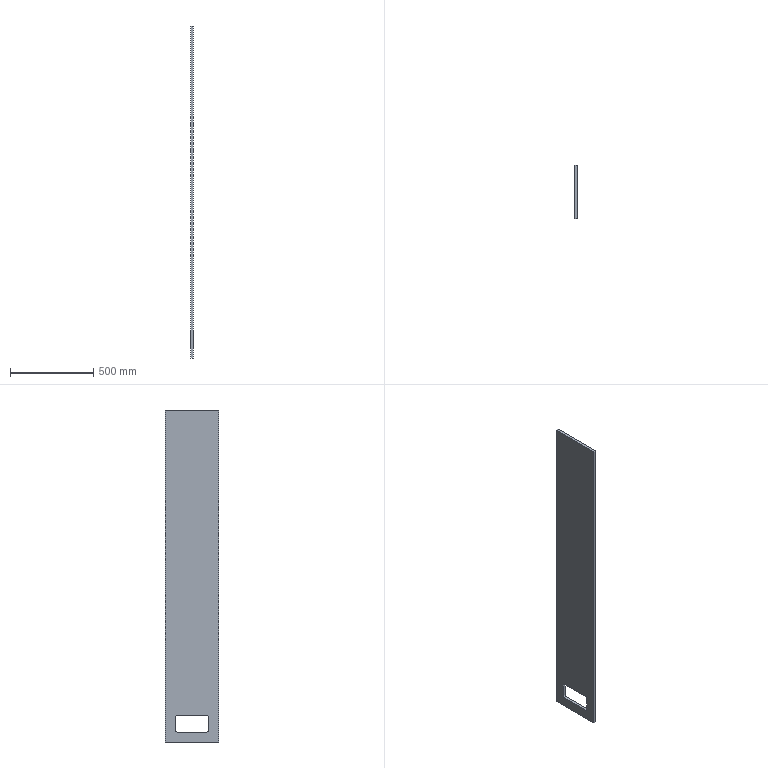Component | NX | CH3404_5-1 | 1 solid | 14 faces | box 16 x 321 x 2000 mm | volume 9953373 mm3 | plane 10 | cylinder 4 | commonest cylinder face diameters 20 x4
STEP:
#1=CARTESIAN_POINT('',(0.,0.,0.));
#2=DIRECTION('',(0.,0.,1.));
#3=DIRECTION('',(1.,0.,0.));
#4=AXIS2_PLACEMENT_3D('',#1,#2,#3);
#5=CARTESIAN_POINT('',(295.,-100.,-155.));
#6=VERTEX_POINT('',#5);
#7=CARTESIAN_POINT('',(295.,-100.,-75.));
#8=VERTEX_POINT('',#7);
#9=CARTESIAN_POINT('',(295.,-100.,-165.));
#10=DIRECTION('',(0.,0.,1.));
#11=VECTOR('',#10,1.);
#12=LINE('',#9,#11);
#13=CARTESIAN_POINT('',(295.,-100.,-165.));
#14=DIRECTION('',(0.,-1.,0.));
#15=DIRECTION('',(0.,0.,-1.));
#16=AXIS2_PLACEMENT_3D('',#13,#14,#15);
#17=PLANE('',#16);
#18=CARTESIAN_POINT('',(0.,0.));
#19=DIRECTION('',(-1.,0.));
#20=VECTOR('',#19,1.);
#21=LINE('',#18,#20);
#22=(GEOMETRIC_REPRESENTATION_CONTEXT(2)PARAMETRIC_REPRESENTATION_CONTEXT()REPRESENTATION_CONTEXT('',''));
#23=DEFINITIONAL_REPRESENTATION('',(#21),#22);
#24=PCURVE('',#17,#23);
#25=CARTESIAN_POINT('',(295.,0.,-225.));
#26=DIRECTION('',(1.,0.,0.));
#27=DIRECTION('',(0.,0.,-1.));
#28=AXIS2_PLACEMENT_3D('',#25,#26,#27);
#29=PLANE('',#28);
#30=CARTESIAN_POINT('',(-60.,-100.));
#31=DIRECTION('',(-1.,0.));
#32=VECTOR('',#31,1.);
#33=LINE('',#30,#32);
#34=(GEOMETRIC_REPRESENTATION_CONTEXT(2)PARAMETRIC_REPRESENTATION_CONTEXT()REPRESENTATION_CONTEXT('',''));
#35=DEFINITIONAL_REPRESENTATION('',(#33),#34);
#36=PCURVE('',#29,#35);
#37=SURFACE_CURVE('',#12,(#24,#36),.PCURVE_S1.);
#38=EDGE_CURVE('',#6,#8,#37,.T.);
#39=ORIENTED_EDGE('',*,*,#38,.F.);
#40=CARTESIAN_POINT('',(279.,-100.,-155.));
#41=VERTEX_POINT('',#40);
#42=CARTESIAN_POINT('',(279.,-100.,-155.));
#43=DIRECTION('',(-1.,0.,0.));
#44=VECTOR('',#43,1.);
#45=LINE('',#42,#44);
#46=CARTESIAN_POINT('',(-10.,-16.));
#47=DIRECTION('',(0.,-1.));
#48=VECTOR('',#47,1.);
#49=LINE('',#46,#48);
#50=(GEOMETRIC_REPRESENTATION_CONTEXT(2)PARAMETRIC_REPRESENTATION_CONTEXT()REPRESENTATION_CONTEXT('',''));
#51=DEFINITIONAL_REPRESENTATION('',(#49),#50);
#52=PCURVE('',#17,#51);
#53=CARTESIAN_POINT('',(295.,-90.,-155.));
#54=DIRECTION('',(1.,0.,0.));
#55=DIRECTION('',(0.,0.,-1.));
#56=AXIS2_PLACEMENT_3D('',#53,#54,#55);
#57=CYLINDRICAL_SURFACE('',#56,10.);
#58=CARTESIAN_POINT('',(4.712,-16.));
#59=DIRECTION('',(0.,-1.));
#60=VECTOR('',#59,1.);
#61=LINE('',#58,#60);
#62=(GEOMETRIC_REPRESENTATION_CONTEXT(2)PARAMETRIC_REPRESENTATION_CONTEXT()REPRESENTATION_CONTEXT('',''));
#63=DEFINITIONAL_REPRESENTATION('',(#61),#62);
#64=PCURVE('',#57,#63);
#65=SURFACE_CURVE('',#45,(#52,#64),.PCURVE_S1.);
#66=EDGE_CURVE('',#6,#41,#65,.T.);
#67=ORIENTED_EDGE('',*,*,#66,.T.);
#68=CARTESIAN_POINT('',(279.,-100.,-75.));
#69=VERTEX_POINT('',#68);
#70=CARTESIAN_POINT('',(279.,-100.,-165.));
#71=DIRECTION('',(0.,0.,1.));
#72=VECTOR('',#71,1.);
#73=LINE('',#70,#72);
#74=CARTESIAN_POINT('',(0.,-16.));
#75=DIRECTION('',(-1.,0.));
#76=VECTOR('',#75,1.);
#77=LINE('',#74,#76);
#78=(GEOMETRIC_REPRESENTATION_CONTEXT(2)PARAMETRIC_REPRESENTATION_CONTEXT()REPRESENTATION_CONTEXT('',''));
#79=DEFINITIONAL_REPRESENTATION('',(#77),#78);
#80=PCURVE('',#17,#79);
#81=CARTESIAN_POINT('',(279.,0.,-225.));
#82=DIRECTION('',(1.,0.,0.));
#83=DIRECTION('',(0.,0.,-1.));
#84=AXIS2_PLACEMENT_3D('',#81,#82,#83);
#85=PLANE('',#84);
#86=CARTESIAN_POINT('',(-60.,-100.));
#87=DIRECTION('',(-1.,0.));
#88=VECTOR('',#87,1.);
#89=LINE('',#86,#88);
#90=(GEOMETRIC_REPRESENTATION_CONTEXT(2)PARAMETRIC_REPRESENTATION_CONTEXT()REPRESENTATION_CONTEXT('',''));
#91=DEFINITIONAL_REPRESENTATION('',(#89),#90);
#92=PCURVE('',#85,#91);
#93=SURFACE_CURVE('',#73,(#80,#92),.PCURVE_S1.);
#94=EDGE_CURVE('',#41,#69,#93,.T.);
#95=ORIENTED_EDGE('',*,*,#94,.T.);
#96=CARTESIAN_POINT('',(295.,-100.,-75.));
#97=DIRECTION('',(1.,0.,0.));
#98=VECTOR('',#97,1.);
#99=LINE('',#96,#98);
#100=CARTESIAN_POINT('',(-90.,0.));
#101=DIRECTION('',(0.,1.));
#102=VECTOR('',#101,1.);
#103=LINE('',#100,#102);
#104=(GEOMETRIC_REPRESENTATION_CONTEXT(2)PARAMETRIC_REPRESENTATION_CONTEXT()REPRESENTATION_CONTEXT('',''));
#105=DEFINITIONAL_REPRESENTATION('',(#103),#104);
#106=PCURVE('',#17,#105);
#107=CARTESIAN_POINT('',(295.,-90.,-75.));
#108=DIRECTION('',(1.,0.,0.));
#109=DIRECTION('',(0.,0.,-1.));
#110=AXIS2_PLACEMENT_3D('',#107,#108,#109);
#111=CYLINDRICAL_SURFACE('',#110,10.);
#112=CARTESIAN_POINT('',(4.712,0.));
#113=DIRECTION('',(0.,1.));
#114=VECTOR('',#113,1.);
#115=LINE('',#112,#114);
#116=(GEOMETRIC_REPRESENTATION_CONTEXT(2)PARAMETRIC_REPRESENTATION_CONTEXT()REPRESENTATION_CONTEXT('',''));
#117=DEFINITIONAL_REPRESENTATION('',(#115),#116);
#118=PCURVE('',#111,#117);
#119=SURFACE_CURVE('',#99,(#106,#118),.PCURVE_S1.);
#120=EDGE_CURVE('',#69,#8,#119,.T.);
#121=ORIENTED_EDGE('',*,*,#120,.T.);
#122=EDGE_LOOP('',(#39,#67,#95,#121));
#123=FACE_BOUND('',#122,.T.);
#124=ADVANCED_FACE('',(#123),#17,.F.);
#125=CARTESIAN_POINT('',(295.,-90.,-65.));
#126=VERTEX_POINT('',#125);
#127=CARTESIAN_POINT('',(295.,90.,-65.));
#128=VERTEX_POINT('',#127);
#129=CARTESIAN_POINT('',(295.,-100.,-65.));
#130=DIRECTION('',(0.,1.,0.));
#131=VECTOR('',#130,1.);
#132=LINE('',#129,#131);
#133=CARTESIAN_POINT('',(295.,-100.,-65.));
#134=DIRECTION('',(0.,0.,1.));
#135=DIRECTION('',(1.,0.,0.));
#136=AXIS2_PLACEMENT_3D('',#133,#134,#135);
#137=PLANE('',#136);
#138=CARTESIAN_POINT('',(0.,0.));
#139=DIRECTION('',(0.,1.));
#140=VECTOR('',#139,1.);
#141=LINE('',#138,#140);
#142=(GEOMETRIC_REPRESENTATION_CONTEXT(2)PARAMETRIC_REPRESENTATION_CONTEXT()REPRESENTATION_CONTEXT('',''));
#143=DEFINITIONAL_REPRESENTATION('',(#141),#142);
#144=PCURVE('',#137,#143);
#145=CARTESIAN_POINT('',(-160.,-100.));
#146=DIRECTION('',(0.,1.));
#147=VECTOR('',#146,1.);
#148=LINE('',#145,#147);
#149=(GEOMETRIC_REPRESENTATION_CONTEXT(2)PARAMETRIC_REPRESENTATION_CONTEXT()REPRESENTATION_CONTEXT('',''));
#150=DEFINITIONAL_REPRESENTATION('',(#148),#149);
#151=PCURVE('',#29,#150);
#152=SURFACE_CURVE('',#132,(#144,#151),.PCURVE_S1.);
#153=EDGE_CURVE('',#126,#128,#152,.T.);
#154=ORIENTED_EDGE('',*,*,#153,.F.);
#155=CARTESIAN_POINT('',(279.,-90.,-65.));
#156=VERTEX_POINT('',#155);
#157=CARTESIAN_POINT('',(279.,-90.,-65.));
#158=DIRECTION('',(-1.,0.,0.));
#159=VECTOR('',#158,1.);
#160=LINE('',#157,#159);
#161=CARTESIAN_POINT('',(-16.,10.));
#162=DIRECTION('',(-1.,0.));
#163=VECTOR('',#162,1.);
#164=LINE('',#161,#163);
#165=(GEOMETRIC_REPRESENTATION_CONTEXT(2)PARAMETRIC_REPRESENTATION_CONTEXT()REPRESENTATION_CONTEXT('',''));
#166=DEFINITIONAL_REPRESENTATION('',(#164),#165);
#167=PCURVE('',#137,#166);
#168=CARTESIAN_POINT('',(3.142,-16.));
#169=DIRECTION('',(0.,-1.));
#170=VECTOR('',#169,1.);
#171=LINE('',#168,#170);
#172=(GEOMETRIC_REPRESENTATION_CONTEXT(2)PARAMETRIC_REPRESENTATION_CONTEXT()REPRESENTATION_CONTEXT('',''));
#173=DEFINITIONAL_REPRESENTATION('',(#171),#172);
#174=PCURVE('',#111,#173);
#175=SURFACE_CURVE('',#160,(#167,#174),.PCURVE_S1.);
#176=EDGE_CURVE('',#126,#156,#175,.T.);
#177=ORIENTED_EDGE('',*,*,#176,.T.);
#178=CARTESIAN_POINT('',(279.,90.,-65.));
#179=VERTEX_POINT('',#178);
#180=CARTESIAN_POINT('',(279.,-100.,-65.));
#181=DIRECTION('',(0.,1.,0.));
#182=VECTOR('',#181,1.);
#183=LINE('',#180,#182);
#184=CARTESIAN_POINT('',(-16.,0.));
#185=DIRECTION('',(0.,1.));
#186=VECTOR('',#185,1.);
#187=LINE('',#184,#186);
#188=(GEOMETRIC_REPRESENTATION_CONTEXT(2)PARAMETRIC_REPRESENTATION_CONTEXT()REPRESENTATION_CONTEXT('',''));
#189=DEFINITIONAL_REPRESENTATION('',(#187),#188);
#190=PCURVE('',#137,#189);
#191=CARTESIAN_POINT('',(-160.,-100.));
#192=DIRECTION('',(0.,1.));
#193=VECTOR('',#192,1.);
#194=LINE('',#191,#193);
#195=(GEOMETRIC_REPRESENTATION_CONTEXT(2)PARAMETRIC_REPRESENTATION_CONTEXT()REPRESENTATION_CONTEXT('',''));
#196=DEFINITIONAL_REPRESENTATION('',(#194),#195);
#197=PCURVE('',#85,#196);
#198=SURFACE_CURVE('',#183,(#190,#197),.PCURVE_S1.);
#199=EDGE_CURVE('',#156,#179,#198,.T.);
#200=ORIENTED_EDGE('',*,*,#199,.T.);
#201=CARTESIAN_POINT('',(295.,90.,-65.));
#202=DIRECTION('',(1.,0.,0.));
#203=VECTOR('',#202,1.);
#204=LINE('',#201,#203);
#205=CARTESIAN_POINT('',(0.,190.));
#206=DIRECTION('',(1.,0.));
#207=VECTOR('',#206,1.);
#208=LINE('',#205,#207);
#209=(GEOMETRIC_REPRESENTATION_CONTEXT(2)PARAMETRIC_REPRESENTATION_CONTEXT()REPRESENTATION_CONTEXT('',''));
#210=DEFINITIONAL_REPRESENTATION('',(#208),#209);
#211=PCURVE('',#137,#210);
#212=CARTESIAN_POINT('',(295.,90.,-75.));
#213=DIRECTION('',(1.,0.,0.));
#214=DIRECTION('',(0.,0.,-1.));
#215=AXIS2_PLACEMENT_3D('',#212,#213,#214);
#216=CYLINDRICAL_SURFACE('',#215,10.);
#217=CARTESIAN_POINT('',(3.142,0.));
#218=DIRECTION('',(0.,1.));
#219=VECTOR('',#218,1.);
#220=LINE('',#217,#219);
#221=(GEOMETRIC_REPRESENTATION_CONTEXT(2)PARAMETRIC_REPRESENTATION_CONTEXT()REPRESENTATION_CONTEXT('',''));
#222=DEFINITIONAL_REPRESENTATION('',(#220),#221);
#223=PCURVE('',#216,#222);
#224=SURFACE_CURVE('',#204,(#211,#223),.PCURVE_S1.);
#225=EDGE_CURVE('',#179,#128,#224,.T.);
#226=ORIENTED_EDGE('',*,*,#225,.T.);
#227=EDGE_LOOP('',(#154,#177,#200,#226));
#228=FACE_BOUND('',#227,.T.);
#229=ADVANCED_FACE('',(#228),#137,.F.);
#230=CARTESIAN_POINT('',(279.,100.,-75.));
#231=VERTEX_POINT('',#230);
#232=CARTESIAN_POINT('',(279.,100.,-155.));
#233=VERTEX_POINT('',#232);
#234=CARTESIAN_POINT('',(279.,100.,-65.));
#235=DIRECTION('',(0.,0.,-1.));
#236=VECTOR('',#235,1.);
#237=LINE('',#234,#236);
#238=CARTESIAN_POINT('',(295.,100.,-65.));
#239=DIRECTION('',(0.,1.,0.));
#240=DIRECTION('',(0.,0.,1.));
#241=AXIS2_PLACEMENT_3D('',#238,#239,#240);
#242=PLANE('',#241);
#243=CARTESIAN_POINT('',(0.,-16.));
#244=DIRECTION('',(-1.,0.));
#245=VECTOR('',#244,1.);
#246=LINE('',#243,#245);
#247=(GEOMETRIC_REPRESENTATION_CONTEXT(2)PARAMETRIC_REPRESENTATION_CONTEXT()REPRESENTATION_CONTEXT('',''));
#248=DEFINITIONAL_REPRESENTATION('',(#246),#247);
#249=PCURVE('',#242,#248);
#250=CARTESIAN_POINT('',(-160.,100.));
#251=DIRECTION('',(1.,0.));
#252=VECTOR('',#251,1.);
#253=LINE('',#250,#252);
#254=(GEOMETRIC_REPRESENTATION_CONTEXT(2)PARAMETRIC_REPRESENTATION_CONTEXT()REPRESENTATION_CONTEXT('',''));
#255=DEFINITIONAL_REPRESENTATION('',(#253),#254);
#256=PCURVE('',#85,#255);
#257=SURFACE_CURVE('',#237,(#249,#256),.PCURVE_S1.);
#258=EDGE_CURVE('',#231,#233,#257,.T.);
#259=ORIENTED_EDGE('',*,*,#258,.T.);
#260=CARTESIAN_POINT('',(295.,100.,-155.));
#261=VERTEX_POINT('',#260);
#262=CARTESIAN_POINT('',(295.,100.,-155.));
#263=DIRECTION('',(1.,0.,0.));
#264=VECTOR('',#263,1.);
#265=LINE('',#262,#264);
#266=CARTESIAN_POINT('',(-90.,0.));
#267=DIRECTION('',(0.,1.));
#268=VECTOR('',#267,1.);
#269=LINE('',#266,#268);
#270=(GEOMETRIC_REPRESENTATION_CONTEXT(2)PARAMETRIC_REPRESENTATION_CONTEXT()REPRESENTATION_CONTEXT('',''));
#271=DEFINITIONAL_REPRESENTATION('',(#269),#270);
#272=PCURVE('',#242,#271);
#273=CARTESIAN_POINT('',(295.,90.,-155.));
#274=DIRECTION('',(1.,0.,0.));
#275=DIRECTION('',(0.,0.,-1.));
#276=AXIS2_PLACEMENT_3D('',#273,#274,#275);
#277=CYLINDRICAL_SURFACE('',#276,10.);
#278=CARTESIAN_POINT('',(1.571,0.));
#279=DIRECTION('',(0.,1.));
#280=VECTOR('',#279,1.);
#281=LINE('',#278,#280);
#282=(GEOMETRIC_REPRESENTATION_CONTEXT(2)PARAMETRIC_REPRESENTATION_CONTEXT()REPRESENTATION_CONTEXT('',''));
#283=DEFINITIONAL_REPRESENTATION('',(#281),#282);
#284=PCURVE('',#277,#283);
#285=SURFACE_CURVE('',#265,(#272,#284),.PCURVE_S1.);
#286=EDGE_CURVE('',#233,#261,#285,.T.);
#287=ORIENTED_EDGE('',*,*,#286,.T.);
#288=CARTESIAN_POINT('',(295.,100.,-75.));
#289=VERTEX_POINT('',#288);
#290=CARTESIAN_POINT('',(295.,100.,-65.));
#291=DIRECTION('',(0.,0.,-1.));
#292=VECTOR('',#291,1.);
#293=LINE('',#290,#292);
#294=CARTESIAN_POINT('',(0.,0.));
#295=DIRECTION('',(-1.,0.));
#296=VECTOR('',#295,1.);
#297=LINE('',#294,#296);
#298=(GEOMETRIC_REPRESENTATION_CONTEXT(2)PARAMETRIC_REPRESENTATION_CONTEXT()REPRESENTATION_CONTEXT('',''));
#299=DEFINITIONAL_REPRESENTATION('',(#297),#298);
#300=PCURVE('',#242,#299);
#301=CARTESIAN_POINT('',(-160.,100.));
#302=DIRECTION('',(1.,0.));
#303=VECTOR('',#302,1.);
#304=LINE('',#301,#303);
#305=(GEOMETRIC_REPRESENTATION_CONTEXT(2)PARAMETRIC_REPRESENTATION_CONTEXT()REPRESENTATION_CONTEXT('',''));
#306=DEFINITIONAL_REPRESENTATION('',(#304),#305);
#307=PCURVE('',#29,#306);
#308=SURFACE_CURVE('',#293,(#300,#307),.PCURVE_S1.);
#309=EDGE_CURVE('',#289,#261,#308,.T.);
#310=ORIENTED_EDGE('',*,*,#309,.F.);
#311=CARTESIAN_POINT('',(279.,100.,-75.));
#312=DIRECTION('',(-1.,0.,0.));
#313=VECTOR('',#312,1.);
#314=LINE('',#311,#313);
#315=CARTESIAN_POINT('',(-10.,-16.));
#316=DIRECTION('',(0.,-1.));
#317=VECTOR('',#316,1.);
#318=LINE('',#315,#317);
#319=(GEOMETRIC_REPRESENTATION_CONTEXT(2)PARAMETRIC_REPRESENTATION_CONTEXT()REPRESENTATION_CONTEXT('',''));
#320=DEFINITIONAL_REPRESENTATION('',(#318),#319);
#321=PCURVE('',#242,#320);
#322=CARTESIAN_POINT('',(1.571,-16.));
#323=DIRECTION('',(0.,-1.));
#324=VECTOR('',#323,1.);
#325=LINE('',#322,#324);
#326=(GEOMETRIC_REPRESENTATION_CONTEXT(2)PARAMETRIC_REPRESENTATION_CONTEXT()REPRESENTATION_CONTEXT('',''));
#327=DEFINITIONAL_REPRESENTATION('',(#325),#326);
#328=PCURVE('',#216,#327);
#329=SURFACE_CURVE('',#314,(#321,#328),.PCURVE_S1.);
#330=EDGE_CURVE('',#289,#231,#329,.T.);
#331=ORIENTED_EDGE('',*,*,#330,.T.);
#332=EDGE_LOOP('',(#259,#287,#310,#331));
#333=FACE_BOUND('',#332,.T.);
#334=ADVANCED_FACE('',(#333),#242,.F.);
#335=CARTESIAN_POINT('',(279.,-160.5,1775.));
#336=VERTEX_POINT('',#335);
#337=CARTESIAN_POINT('',(279.,-160.5,-225.));
#338=VERTEX_POINT('',#337);
#339=CARTESIAN_POINT('',(279.,-160.5,1775.));
#340=DIRECTION('',(0.,-0.,-1.));
#341=VECTOR('',#340,1.);
#342=LINE('',#339,#341);
#343=CARTESIAN_POINT('',(295.,-160.5,1775.));
#344=DIRECTION('',(0.,1.,-0.));
#345=DIRECTION('',(0.,0.,1.));
#346=AXIS2_PLACEMENT_3D('',#343,#344,#345);
#347=PLANE('',#346);
#348=CARTESIAN_POINT('',(0.,-16.));
#349=DIRECTION('',(-1.,0.));
#350=VECTOR('',#349,1.);
#351=LINE('',#348,#350);
#352=(GEOMETRIC_REPRESENTATION_CONTEXT(2)PARAMETRIC_REPRESENTATION_CONTEXT()REPRESENTATION_CONTEXT('',''));
#353=DEFINITIONAL_REPRESENTATION('',(#351),#352);
#354=PCURVE('',#347,#353);
#355=CARTESIAN_POINT('',(-2000.,-160.5));
#356=DIRECTION('',(1.,-0.));
#357=VECTOR('',#356,1.);
#358=LINE('',#355,#357);
#359=(GEOMETRIC_REPRESENTATION_CONTEXT(2)PARAMETRIC_REPRESENTATION_CONTEXT()REPRESENTATION_CONTEXT('',''));
#360=DEFINITIONAL_REPRESENTATION('',(#358),#359);
#361=PCURVE('',#85,#360);
#362=SURFACE_CURVE('',#342,(#354,#361),.PCURVE_S1.);
#363=EDGE_CURVE('',#336,#338,#362,.T.);
#364=ORIENTED_EDGE('',*,*,#363,.T.);
#365=CARTESIAN_POINT('',(295.,-160.5,-225.));
#366=VERTEX_POINT('',#365);
#367=CARTESIAN_POINT('',(295.,-160.5,-225.));
#368=DIRECTION('',(-1.,0.,0.));
#369=VECTOR('',#368,1.);
#370=LINE('',#367,#369);
#371=CARTESIAN_POINT('',(-2000.,0.));
#372=DIRECTION('',(0.,-1.));
#373=VECTOR('',#372,1.);
#374=LINE('',#371,#373);
#375=(GEOMETRIC_REPRESENTATION_CONTEXT(2)PARAMETRIC_REPRESENTATION_CONTEXT()REPRESENTATION_CONTEXT('',''));
#376=DEFINITIONAL_REPRESENTATION('',(#374),#375);
#377=PCURVE('',#347,#376);
#378=CARTESIAN_POINT('',(295.,-160.5,-225.));
#379=DIRECTION('',(0.,0.,1.));
#380=DIRECTION('',(1.,0.,0.));
#381=AXIS2_PLACEMENT_3D('',#378,#379,#380);
#382=PLANE('',#381);
#383=CARTESIAN_POINT('',(0.,0.));
#384=DIRECTION('',(-1.,0.));
#385=VECTOR('',#384,1.);
#386=LINE('',#383,#385);
#387=(GEOMETRIC_REPRESENTATION_CONTEXT(2)PARAMETRIC_REPRESENTATION_CONTEXT()REPRESENTATION_CONTEXT('',''));
#388=DEFINITIONAL_REPRESENTATION('',(#386),#387);
#389=PCURVE('',#382,#388);
#390=SURFACE_CURVE('',#370,(#377,#389),.PCURVE_S1.);
#391=EDGE_CURVE('',#366,#338,#390,.T.);
#392=ORIENTED_EDGE('',*,*,#391,.F.);
#393=CARTESIAN_POINT('',(295.,-160.5,1775.));
#394=VERTEX_POINT('',#393);
#395=CARTESIAN_POINT('',(295.,-160.5,1775.));
#396=DIRECTION('',(0.,-0.,-1.));
#397=VECTOR('',#396,1.);
#398=LINE('',#395,#397);
#399=CARTESIAN_POINT('',(0.,0.));
#400=DIRECTION('',(-1.,0.));
#401=VECTOR('',#400,1.);
#402=LINE('',#399,#401);
#403=(GEOMETRIC_REPRESENTATION_CONTEXT(2)PARAMETRIC_REPRESENTATION_CONTEXT()REPRESENTATION_CONTEXT('',''));
#404=DEFINITIONAL_REPRESENTATION('',(#402),#403);
#405=PCURVE('',#347,#404);
#406=CARTESIAN_POINT('',(-2000.,-160.5));
#407=DIRECTION('',(1.,-0.));
#408=VECTOR('',#407,1.);
#409=LINE('',#406,#408);
#410=(GEOMETRIC_REPRESENTATION_CONTEXT(2)PARAMETRIC_REPRESENTATION_CONTEXT()REPRESENTATION_CONTEXT('',''));
#411=DEFINITIONAL_REPRESENTATION('',(#409),#410);
#412=PCURVE('',#29,#411);
#413=SURFACE_CURVE('',#398,(#405,#412),.PCURVE_S1.);
#414=EDGE_CURVE('',#394,#366,#413,.T.);
#415=ORIENTED_EDGE('',*,*,#414,.F.);
#416=CARTESIAN_POINT('',(295.,-160.5,1775.));
#417=DIRECTION('',(-1.,0.,0.));
#418=VECTOR('',#417,1.);
#419=LINE('',#416,#418);
#420=CARTESIAN_POINT('',(0.,0.));
#421=DIRECTION('',(0.,-1.));
#422=VECTOR('',#421,1.);
#423=LINE('',#420,#422);
#424=(GEOMETRIC_REPRESENTATION_CONTEXT(2)PARAMETRIC_REPRESENTATION_CONTEXT()REPRESENTATION_CONTEXT('',''));
#425=DEFINITIONAL_REPRESENTATION('',(#423),#424);
#426=PCURVE('',#347,#425);
#427=CARTESIAN_POINT('',(295.,160.5,1775.));
#428=DIRECTION('',(0.,0.,-1.));
#429=DIRECTION('',(-1.,0.,0.));
#430=AXIS2_PLACEMENT_3D('',#427,#428,#429);
#431=PLANE('',#430);
#432=CARTESIAN_POINT('',(0.,-321.));
#433=DIRECTION('',(1.,0.));
#434=VECTOR('',#433,1.);
#435=LINE('',#432,#434);
#436=(GEOMETRIC_REPRESENTATION_CONTEXT(2)PARAMETRIC_REPRESENTATION_CONTEXT()REPRESENTATION_CONTEXT('',''));
#437=DEFINITIONAL_REPRESENTATION('',(#435),#436);
#438=PCURVE('',#431,#437);
#439=SURFACE_CURVE('',#419,(#426,#438),.PCURVE_S1.);
#440=EDGE_CURVE('',#394,#336,#439,.T.);
#441=ORIENTED_EDGE('',*,*,#440,.T.);
#442=EDGE_LOOP('',(#364,#392,#415,#441));
#443=FACE_BOUND('',#442,.T.);
#444=ADVANCED_FACE('',(#443),#347,.F.);
#445=CARTESIAN_POINT('',(279.,160.5,-225.));
#446=VERTEX_POINT('',#445);
#447=CARTESIAN_POINT('',(279.,-160.5,-225.));
#448=DIRECTION('',(0.,1.,0.));
#449=VECTOR('',#448,1.);
#450=LINE('',#447,#449);
#451=CARTESIAN_POINT('',(-16.,0.));
#452=DIRECTION('',(0.,1.));
#453=VECTOR('',#452,1.);
#454=LINE('',#451,#453);
#455=(GEOMETRIC_REPRESENTATION_CONTEXT(2)PARAMETRIC_REPRESENTATION_CONTEXT()REPRESENTATION_CONTEXT('',''));
#456=DEFINITIONAL_REPRESENTATION('',(#454),#455);
#457=PCURVE('',#382,#456);
#458=CARTESIAN_POINT('',(0.,-160.5));
#459=DIRECTION('',(0.,1.));
#460=VECTOR('',#459,1.);
#461=LINE('',#458,#460);
#462=(GEOMETRIC_REPRESENTATION_CONTEXT(2)PARAMETRIC_REPRESENTATION_CONTEXT()REPRESENTATION_CONTEXT('',''));
#463=DEFINITIONAL_REPRESENTATION('',(#461),#462);
#464=PCURVE('',#85,#463);
#465=SURFACE_CURVE('',#450,(#457,#464),.PCURVE_S1.);
#466=EDGE_CURVE('',#338,#446,#465,.T.);
#467=ORIENTED_EDGE('',*,*,#466,.T.);
#468=CARTESIAN_POINT('',(295.,160.5,-225.));
#469=VERTEX_POINT('',#468);
#470=CARTESIAN_POINT('',(295.,160.5,-225.));
#471=DIRECTION('',(-1.,0.,0.));
#472=VECTOR('',#471,1.);
#473=LINE('',#470,#472);
#474=CARTESIAN_POINT('',(0.,321.));
#475=DIRECTION('',(-1.,0.));
#476=VECTOR('',#475,1.);
#477=LINE('',#474,#476);
#478=(GEOMETRIC_REPRESENTATION_CONTEXT(2)PARAMETRIC_REPRESENTATION_CONTEXT()REPRESENTATION_CONTEXT('',''));
#479=DEFINITIONAL_REPRESENTATION('',(#477),#478);
#480=PCURVE('',#382,#479);
#481=CARTESIAN_POINT('',(295.,160.5,-225.));
#482=DIRECTION('',(0.,-1.,-0.));
#483=DIRECTION('',(0.,0.,-1.));
#484=AXIS2_PLACEMENT_3D('',#481,#482,#483);
#485=PLANE('',#484);
#486=CARTESIAN_POINT('',(0.,0.));
#487=DIRECTION('',(0.,-1.));
#488=VECTOR('',#487,1.);
#489=LINE('',#486,#488);
#490=(GEOMETRIC_REPRESENTATION_CONTEXT(2)PARAMETRIC_REPRESENTATION_CONTEXT()REPRESENTATION_CONTEXT('',''));
#491=DEFINITIONAL_REPRESENTATION('',(#489),#490);
#492=PCURVE('',#485,#491);
#493=SURFACE_CURVE('',#473,(#480,#492),.PCURVE_S1.);
#494=EDGE_CURVE('',#469,#446,#493,.T.);
#495=ORIENTED_EDGE('',*,*,#494,.F.);
#496=CARTESIAN_POINT('',(295.,-160.5,-225.));
#497=DIRECTION('',(0.,1.,0.));
#498=VECTOR('',#497,1.);
#499=LINE('',#496,#498);
#500=CARTESIAN_POINT('',(0.,0.));
#501=DIRECTION('',(0.,1.));
#502=VECTOR('',#501,1.);
#503=LINE('',#500,#502);
#504=(GEOMETRIC_REPRESENTATION_CONTEXT(2)PARAMETRIC_REPRESENTATION_CONTEXT()REPRESENTATION_CONTEXT('',''));
#505=DEFINITIONAL_REPRESENTATION('',(#503),#504);
#506=PCURVE('',#382,#505);
#507=CARTESIAN_POINT('',(0.,-160.5));
#508=DIRECTION('',(0.,1.));
#509=VECTOR('',#508,1.);
#510=LINE('',#507,#509);
#511=(GEOMETRIC_REPRESENTATION_CONTEXT(2)PARAMETRIC_REPRESENTATION_CONTEXT()REPRESENTATION_CONTEXT('',''));
#512=DEFINITIONAL_REPRESENTATION('',(#510),#511);
#513=PCURVE('',#29,#512);
#514=SURFACE_CURVE('',#499,(#506,#513),.PCURVE_S1.);
#515=EDGE_CURVE('',#366,#469,#514,.T.);
#516=ORIENTED_EDGE('',*,*,#515,.F.);
#517=ORIENTED_EDGE('',*,*,#391,.T.);
#518=EDGE_LOOP('',(#467,#495,#516,#517));
#519=FACE_BOUND('',#518,.T.);
#520=ADVANCED_FACE('',(#519),#382,.F.);
#521=CARTESIAN_POINT('',(279.,160.5,1775.));
#522=VERTEX_POINT('',#521);
#523=CARTESIAN_POINT('',(279.,160.5,-225.));
#524=DIRECTION('',(0.,-0.,1.));
#525=VECTOR('',#524,1.);
#526=LINE('',#523,#525);
#527=CARTESIAN_POINT('',(0.,-16.));
#528=DIRECTION('',(-1.,0.));
#529=VECTOR('',#528,1.);
#530=LINE('',#527,#529);
#531=(GEOMETRIC_REPRESENTATION_CONTEXT(2)PARAMETRIC_REPRESENTATION_CONTEXT()REPRESENTATION_CONTEXT('',''));
#532=DEFINITIONAL_REPRESENTATION('',(#530),#531);
#533=PCURVE('',#485,#532);
#534=CARTESIAN_POINT('',(0.,160.5));
#535=DIRECTION('',(-1.,-0.));
#536=VECTOR('',#535,1.);
#537=LINE('',#534,#536);
#538=(GEOMETRIC_REPRESENTATION_CONTEXT(2)PARAMETRIC_REPRESENTATION_CONTEXT()REPRESENTATION_CONTEXT('',''));
#539=DEFINITIONAL_REPRESENTATION('',(#537),#538);
#540=PCURVE('',#85,#539);
#541=SURFACE_CURVE('',#526,(#533,#540),.PCURVE_S1.);
#542=EDGE_CURVE('',#446,#522,#541,.T.);
#543=ORIENTED_EDGE('',*,*,#542,.T.);
#544=CARTESIAN_POINT('',(295.,160.5,1775.));
#545=VERTEX_POINT('',#544);
#546=CARTESIAN_POINT('',(295.,160.5,1775.));
#547=DIRECTION('',(-1.,0.,0.));
#548=VECTOR('',#547,1.);
#549=LINE('',#546,#548);
#550=CARTESIAN_POINT('',(-2000.,0.));
#551=DIRECTION('',(0.,-1.));
#552=VECTOR('',#551,1.);
#553=LINE('',#550,#552);
#554=(GEOMETRIC_REPRESENTATION_CONTEXT(2)PARAMETRIC_REPRESENTATION_CONTEXT()REPRESENTATION_CONTEXT('',''));
#555=DEFINITIONAL_REPRESENTATION('',(#553),#554);
#556=PCURVE('',#485,#555);
#557=CARTESIAN_POINT('',(0.,0.));
#558=DIRECTION('',(1.,0.));
#559=VECTOR('',#558,1.);
#560=LINE('',#557,#559);
#561=(GEOMETRIC_REPRESENTATION_CONTEXT(2)PARAMETRIC_REPRESENTATION_CONTEXT()REPRESENTATION_CONTEXT('',''));
#562=DEFINITIONAL_REPRESENTATION('',(#560),#561);
#563=PCURVE('',#431,#562);
#564=SURFACE_CURVE('',#549,(#556,#563),.PCURVE_S1.);
#565=EDGE_CURVE('',#545,#522,#564,.T.);
#566=ORIENTED_EDGE('',*,*,#565,.F.);
#567=CARTESIAN_POINT('',(295.,160.5,-225.));
#568=DIRECTION('',(0.,-0.,1.));
#569=VECTOR('',#568,1.);
#570=LINE('',#567,#569);
#571=CARTESIAN_POINT('',(0.,0.));
#572=DIRECTION('',(-1.,0.));
#573=VECTOR('',#572,1.);
#574=LINE('',#571,#573);
#575=(GEOMETRIC_REPRESENTATION_CONTEXT(2)PARAMETRIC_REPRESENTATION_CONTEXT()REPRESENTATION_CONTEXT('',''));
#576=DEFINITIONAL_REPRESENTATION('',(#574),#575);
#577=PCURVE('',#485,#576);
#578=CARTESIAN_POINT('',(0.,160.5));
#579=DIRECTION('',(-1.,-0.));
#580=VECTOR('',#579,1.);
#581=LINE('',#578,#580);
#582=(GEOMETRIC_REPRESENTATION_CONTEXT(2)PARAMETRIC_REPRESENTATION_CONTEXT()REPRESENTATION_CONTEXT('',''));
#583=DEFINITIONAL_REPRESENTATION('',(#581),#582);
#584=PCURVE('',#29,#583);
#585=SURFACE_CURVE('',#570,(#577,#584),.PCURVE_S1.);
#586=EDGE_CURVE('',#469,#545,#585,.T.);
#587=ORIENTED_EDGE('',*,*,#586,.F.);
#588=ORIENTED_EDGE('',*,*,#494,.T.);
#589=EDGE_LOOP('',(#543,#566,#587,#588));
#590=FACE_BOUND('',#589,.T.);
#591=ADVANCED_FACE('',(#590),#485,.F.);
#592=CARTESIAN_POINT('',(279.,160.5,1775.));
#593=DIRECTION('',(0.,-1.,0.));
#594=VECTOR('',#593,1.);
#595=LINE('',#592,#594);
#596=CARTESIAN_POINT('',(16.,0.));
#597=DIRECTION('',(0.,-1.));
#598=VECTOR('',#597,1.);
#599=LINE('',#596,#598);
#600=(GEOMETRIC_REPRESENTATION_CONTEXT(2)PARAMETRIC_REPRESENTATION_CONTEXT()REPRESENTATION_CONTEXT('',''));
#601=DEFINITIONAL_REPRESENTATION('',(#599),#600);
#602=PCURVE('',#431,#601);
#603=CARTESIAN_POINT('',(-2000.,160.5));
#604=DIRECTION('',(0.,-1.));
#605=VECTOR('',#604,1.);
#606=LINE('',#603,#605);
#607=(GEOMETRIC_REPRESENTATION_CONTEXT(2)PARAMETRIC_REPRESENTATION_CONTEXT()REPRESENTATION_CONTEXT('',''));
#608=DEFINITIONAL_REPRESENTATION('',(#606),#607);
#609=PCURVE('',#85,#608);
#610=SURFACE_CURVE('',#595,(#602,#609),.PCURVE_S1.);
#611=EDGE_CURVE('',#522,#336,#610,.T.);
#612=ORIENTED_EDGE('',*,*,#611,.T.);
#613=ORIENTED_EDGE('',*,*,#440,.F.);
#614=CARTESIAN_POINT('',(295.,160.5,1775.));
#615=DIRECTION('',(0.,-1.,0.));
#616=VECTOR('',#615,1.);
#617=LINE('',#614,#616);
#618=CARTESIAN_POINT('',(0.,0.));
#619=DIRECTION('',(0.,-1.));
#620=VECTOR('',#619,1.);
#621=LINE('',#618,#620);
#622=(GEOMETRIC_REPRESENTATION_CONTEXT(2)PARAMETRIC_REPRESENTATION_CONTEXT()REPRESENTATION_CONTEXT('',''));
#623=DEFINITIONAL_REPRESENTATION('',(#621),#622);
#624=PCURVE('',#431,#623);
#625=CARTESIAN_POINT('',(-2000.,160.5));
#626=DIRECTION('',(0.,-1.));
#627=VECTOR('',#626,1.);
#628=LINE('',#625,#627);
#629=(GEOMETRIC_REPRESENTATION_CONTEXT(2)PARAMETRIC_REPRESENTATION_CONTEXT()REPRESENTATION_CONTEXT('',''));
#630=DEFINITIONAL_REPRESENTATION('',(#628),#629);
#631=PCURVE('',#29,#630);
#632=SURFACE_CURVE('',#617,(#624,#631),.PCURVE_S1.);
#633=EDGE_CURVE('',#545,#394,#632,.T.);
#634=ORIENTED_EDGE('',*,*,#633,.F.);
#635=ORIENTED_EDGE('',*,*,#565,.T.);
#636=EDGE_LOOP('',(#612,#613,#634,#635));
#637=FACE_BOUND('',#636,.T.);
#638=ADVANCED_FACE('',(#637),#431,.F.);
#639=CARTESIAN_POINT('',(295.,90.,-165.));
#640=VERTEX_POINT('',#639);
#641=CARTESIAN_POINT('',(295.,-90.,-165.));
#642=VERTEX_POINT('',#641);
#643=CARTESIAN_POINT('',(295.,100.,-165.));
#644=DIRECTION('',(0.,-1.,0.));
#645=VECTOR('',#644,1.);
#646=LINE('',#643,#645);
#647=CARTESIAN_POINT('',(295.,100.,-165.));
#648=DIRECTION('',(0.,0.,-1.));
#649=DIRECTION('',(-1.,0.,0.));
#650=AXIS2_PLACEMENT_3D('',#647,#648,#649);
#651=PLANE('',#650);
#652=CARTESIAN_POINT('',(0.,0.));
#653=DIRECTION('',(0.,-1.));
#654=VECTOR('',#653,1.);
#655=LINE('',#652,#654);
#656=(GEOMETRIC_REPRESENTATION_CONTEXT(2)PARAMETRIC_REPRESENTATION_CONTEXT()REPRESENTATION_CONTEXT('',''));
#657=DEFINITIONAL_REPRESENTATION('',(#655),#656);
#658=PCURVE('',#651,#657);
#659=CARTESIAN_POINT('',(-60.,100.));
#660=DIRECTION('',(0.,-1.));
#661=VECTOR('',#660,1.);
#662=LINE('',#659,#661);
#663=(GEOMETRIC_REPRESENTATION_CONTEXT(2)PARAMETRIC_REPRESENTATION_CONTEXT()REPRESENTATION_CONTEXT('',''));
#664=DEFINITIONAL_REPRESENTATION('',(#662),#663);
#665=PCURVE('',#29,#664);
#666=SURFACE_CURVE('',#646,(#658,#665),.PCURVE_S1.);
#667=EDGE_CURVE('',#640,#642,#666,.T.);
#668=ORIENTED_EDGE('',*,*,#667,.F.);
#669=CARTESIAN_POINT('',(279.,90.,-165.));
#670=VERTEX_POINT('',#669);
#671=CARTESIAN_POINT('',(279.,90.,-165.));
#672=DIRECTION('',(-1.,0.,0.));
#673=VECTOR('',#672,1.);
#674=LINE('',#671,#673);
#675=CARTESIAN_POINT('',(16.,-10.));
#676=DIRECTION('',(1.,0.));
#677=VECTOR('',#676,1.);
#678=LINE('',#675,#677);
#679=(GEOMETRIC_REPRESENTATION_CONTEXT(2)PARAMETRIC_REPRESENTATION_CONTEXT()REPRESENTATION_CONTEXT('',''));
#680=DEFINITIONAL_REPRESENTATION('',(#678),#679);
#681=PCURVE('',#651,#680);
#682=CARTESIAN_POINT('',(0.,-16.));
#683=DIRECTION('',(0.,-1.));
#684=VECTOR('',#683,1.);
#685=LINE('',#682,#684);
#686=(GEOMETRIC_REPRESENTATION_CONTEXT(2)PARAMETRIC_REPRESENTATION_CONTEXT()REPRESENTATION_CONTEXT('',''));
#687=DEFINITIONAL_REPRESENTATION('',(#685),#686);
#688=PCURVE('',#277,#687);
#689=SURFACE_CURVE('',#674,(#681,#688),.PCURVE_S1.);
#690=EDGE_CURVE('',#640,#670,#689,.T.);
#691=ORIENTED_EDGE('',*,*,#690,.T.);
#692=CARTESIAN_POINT('',(279.,-90.,-165.));
#693=VERTEX_POINT('',#692);
#694=CARTESIAN_POINT('',(279.,100.,-165.));
#695=DIRECTION('',(0.,-1.,0.));
#696=VECTOR('',#695,1.);
#697=LINE('',#694,#696);
#698=CARTESIAN_POINT('',(16.,0.));
#699=DIRECTION('',(0.,-1.));
#700=VECTOR('',#699,1.);
#701=LINE('',#698,#700);
#702=(GEOMETRIC_REPRESENTATION_CONTEXT(2)PARAMETRIC_REPRESENTATION_CONTEXT()REPRESENTATION_CONTEXT('',''));
#703=DEFINITIONAL_REPRESENTATION('',(#701),#702);
#704=PCURVE('',#651,#703);
#705=CARTESIAN_POINT('',(-60.,100.));
#706=DIRECTION('',(0.,-1.));
#707=VECTOR('',#706,1.);
#708=LINE('',#705,#707);
#709=(GEOMETRIC_REPRESENTATION_CONTEXT(2)PARAMETRIC_REPRESENTATION_CONTEXT()REPRESENTATION_CONTEXT('',''));
#710=DEFINITIONAL_REPRESENTATION('',(#708),#709);
#711=PCURVE('',#85,#710);
#712=SURFACE_CURVE('',#697,(#704,#711),.PCURVE_S1.);
#713=EDGE_CURVE('',#670,#693,#712,.T.);
#714=ORIENTED_EDGE('',*,*,#713,.T.);
#715=CARTESIAN_POINT('',(295.,-90.,-165.));
#716=DIRECTION('',(1.,0.,0.));
#717=VECTOR('',#716,1.);
#718=LINE('',#715,#717);
#719=CARTESIAN_POINT('',(0.,-190.));
#720=DIRECTION('',(-1.,0.));
#721=VECTOR('',#720,1.);
#722=LINE('',#719,#721);
#723=(GEOMETRIC_REPRESENTATION_CONTEXT(2)PARAMETRIC_REPRESENTATION_CONTEXT()REPRESENTATION_CONTEXT('',''));
#724=DEFINITIONAL_REPRESENTATION('',(#722),#723);
#725=PCURVE('',#651,#724);
#726=CARTESIAN_POINT('',(6.283,0.));
#727=DIRECTION('',(0.,1.));
#728=VECTOR('',#727,1.);
#729=LINE('',#726,#728);
#730=(GEOMETRIC_REPRESENTATION_CONTEXT(2)PARAMETRIC_REPRESENTATION_CONTEXT()REPRESENTATION_CONTEXT('',''));
#731=DEFINITIONAL_REPRESENTATION('',(#729),#730);
#732=PCURVE('',#57,#731);
#733=SURFACE_CURVE('',#718,(#725,#732),.PCURVE_S1.);
#734=EDGE_CURVE('',#693,#642,#733,.T.);
#735=ORIENTED_EDGE('',*,*,#734,.T.);
#736=EDGE_LOOP('',(#668,#691,#714,#735));
#737=FACE_BOUND('',#736,.T.);
#738=ADVANCED_FACE('',(#737),#651,.F.);
#739=ORIENTED_EDGE('',*,*,#414,.T.);
#740=ORIENTED_EDGE('',*,*,#515,.T.);
#741=ORIENTED_EDGE('',*,*,#586,.T.);
#742=ORIENTED_EDGE('',*,*,#633,.T.);
#743=EDGE_LOOP('',(#739,#740,#741,#742));
#744=FACE_BOUND('',#743,.T.);
#745=ORIENTED_EDGE('',*,*,#667,.T.);
#746=CARTESIAN_POINT('',(295.,-90.,-155.));
#747=DIRECTION('',(-1.,0.,0.));
#748=DIRECTION('',(0.,0.,-1.));
#749=AXIS2_PLACEMENT_3D('',#746,#747,#748);
#750=CIRCLE('',#749,10.);
#751=CARTESIAN_POINT('',(-60.,-90.));
#752=CARTESIAN_POINT('',(-60.,-107.321));
#753=CARTESIAN_POINT('',(-75.,-98.66));
#754=CARTESIAN_POINT('',(-90.,-90.));
#755=CARTESIAN_POINT('',(-75.,-81.34));
#756=CARTESIAN_POINT('',(-60.,-72.679));
#757=CARTESIAN_POINT('',(-60.,-90.));
#758=(BOUNDED_CURVE()B_SPLINE_CURVE(2,(#751,#752,#753,#754,#755,#756,#757),.UNSPECIFIED.,.T.,.F.)B_SPLINE_CURVE_WITH_KNOTS((1,2,2,2,2,1),(-2.094,0.,2.094,4.189,6.283,8.378),.UNSPECIFIED.)CURVE()GEOMETRIC_REPRESENTATION_ITEM()RATIONAL_B_SPLINE_CURVE((1.,0.5,1.,0.5,1.,0.5,1.))REPRESENTATION_ITEM(''));
#759=(GEOMETRIC_REPRESENTATION_CONTEXT(2)PARAMETRIC_REPRESENTATION_CONTEXT()REPRESENTATION_CONTEXT('',''));
#760=DEFINITIONAL_REPRESENTATION('',(#758),#759);
#761=PCURVE('',#29,#760);
#762=CARTESIAN_POINT('',(6.283,0.));
#763=DIRECTION('',(-1.,0.));
#764=VECTOR('',#763,1.);
#765=LINE('',#762,#764);
#766=(GEOMETRIC_REPRESENTATION_CONTEXT(2)PARAMETRIC_REPRESENTATION_CONTEXT()REPRESENTATION_CONTEXT('',''));
#767=DEFINITIONAL_REPRESENTATION('',(#765),#766);
#768=PCURVE('',#57,#767);
#769=SURFACE_CURVE('',#750,(#761,#768),.PCURVE_S1.);
#770=EDGE_CURVE('',#642,#6,#769,.T.);
#771=ORIENTED_EDGE('',*,*,#770,.T.);
#772=ORIENTED_EDGE('',*,*,#38,.T.);
#773=CARTESIAN_POINT('',(295.,-90.,-75.));
#774=DIRECTION('',(-1.,0.,0.));
#775=DIRECTION('',(0.,0.,-1.));
#776=AXIS2_PLACEMENT_3D('',#773,#774,#775);
#777=CIRCLE('',#776,10.);
#778=CARTESIAN_POINT('',(-140.,-90.));
#779=CARTESIAN_POINT('',(-140.,-107.321));
#780=CARTESIAN_POINT('',(-155.,-98.66));
#781=CARTESIAN_POINT('',(-170.,-90.));
#782=CARTESIAN_POINT('',(-155.,-81.34));
#783=CARTESIAN_POINT('',(-140.,-72.679));
#784=CARTESIAN_POINT('',(-140.,-90.));
#785=(BOUNDED_CURVE()B_SPLINE_CURVE(2,(#778,#779,#780,#781,#782,#783,#784),.UNSPECIFIED.,.T.,.F.)B_SPLINE_CURVE_WITH_KNOTS((1,2,2,2,2,1),(-2.094,0.,2.094,4.189,6.283,8.378),.UNSPECIFIED.)CURVE()GEOMETRIC_REPRESENTATION_ITEM()RATIONAL_B_SPLINE_CURVE((1.,0.5,1.,0.5,1.,0.5,1.))REPRESENTATION_ITEM(''));
#786=(GEOMETRIC_REPRESENTATION_CONTEXT(2)PARAMETRIC_REPRESENTATION_CONTEXT()REPRESENTATION_CONTEXT('',''));
#787=DEFINITIONAL_REPRESENTATION('',(#785),#786);
#788=PCURVE('',#29,#787);
#789=CARTESIAN_POINT('',(6.283,0.));
#790=DIRECTION('',(-1.,0.));
#791=VECTOR('',#790,1.);
#792=LINE('',#789,#791);
#793=(GEOMETRIC_REPRESENTATION_CONTEXT(2)PARAMETRIC_REPRESENTATION_CONTEXT()REPRESENTATION_CONTEXT('',''));
#794=DEFINITIONAL_REPRESENTATION('',(#792),#793);
#795=PCURVE('',#111,#794);
#796=SURFACE_CURVE('',#777,(#788,#795),.PCURVE_S1.);
#797=EDGE_CURVE('',#8,#126,#796,.T.);
#798=ORIENTED_EDGE('',*,*,#797,.T.);
#799=ORIENTED_EDGE('',*,*,#153,.T.);
#800=CARTESIAN_POINT('',(295.,90.,-75.));
#801=DIRECTION('',(-1.,0.,0.));
#802=DIRECTION('',(0.,0.,-1.));
#803=AXIS2_PLACEMENT_3D('',#800,#801,#802);
#804=CIRCLE('',#803,10.);
#805=CARTESIAN_POINT('',(-140.,90.));
#806=CARTESIAN_POINT('',(-140.,72.679));
#807=CARTESIAN_POINT('',(-155.,81.34));
#808=CARTESIAN_POINT('',(-170.,90.));
#809=CARTESIAN_POINT('',(-155.,98.66));
#810=CARTESIAN_POINT('',(-140.,107.321));
#811=CARTESIAN_POINT('',(-140.,90.));
#812=(BOUNDED_CURVE()B_SPLINE_CURVE(2,(#805,#806,#807,#808,#809,#810,#811),.UNSPECIFIED.,.T.,.F.)B_SPLINE_CURVE_WITH_KNOTS((1,2,2,2,2,1),(-2.094,0.,2.094,4.189,6.283,8.378),.UNSPECIFIED.)CURVE()GEOMETRIC_REPRESENTATION_ITEM()RATIONAL_B_SPLINE_CURVE((1.,0.5,1.,0.5,1.,0.5,1.))REPRESENTATION_ITEM(''));
#813=(GEOMETRIC_REPRESENTATION_CONTEXT(2)PARAMETRIC_REPRESENTATION_CONTEXT()REPRESENTATION_CONTEXT('',''));
#814=DEFINITIONAL_REPRESENTATION('',(#812),#813);
#815=PCURVE('',#29,#814);
#816=CARTESIAN_POINT('',(6.283,0.));
#817=DIRECTION('',(-1.,0.));
#818=VECTOR('',#817,1.);
#819=LINE('',#816,#818);
#820=(GEOMETRIC_REPRESENTATION_CONTEXT(2)PARAMETRIC_REPRESENTATION_CONTEXT()REPRESENTATION_CONTEXT('',''));
#821=DEFINITIONAL_REPRESENTATION('',(#819),#820);
#822=PCURVE('',#216,#821);
#823=SURFACE_CURVE('',#804,(#815,#822),.PCURVE_S1.);
#824=EDGE_CURVE('',#128,#289,#823,.T.);
#825=ORIENTED_EDGE('',*,*,#824,.T.);
#826=ORIENTED_EDGE('',*,*,#309,.T.);
#827=CARTESIAN_POINT('',(295.,90.,-155.));
#828=DIRECTION('',(-1.,0.,0.));
#829=DIRECTION('',(0.,0.,-1.));
#830=AXIS2_PLACEMENT_3D('',#827,#828,#829);
#831=CIRCLE('',#830,10.);
#832=CARTESIAN_POINT('',(-60.,90.));
#833=CARTESIAN_POINT('',(-60.,72.679));
#834=CARTESIAN_POINT('',(-75.,81.34));
#835=CARTESIAN_POINT('',(-90.,90.));
#836=CARTESIAN_POINT('',(-75.,98.66));
#837=CARTESIAN_POINT('',(-60.,107.321));
#838=CARTESIAN_POINT('',(-60.,90.));
#839=(BOUNDED_CURVE()B_SPLINE_CURVE(2,(#832,#833,#834,#835,#836,#837,#838),.UNSPECIFIED.,.T.,.F.)B_SPLINE_CURVE_WITH_KNOTS((1,2,2,2,2,1),(-2.094,0.,2.094,4.189,6.283,8.378),.UNSPECIFIED.)CURVE()GEOMETRIC_REPRESENTATION_ITEM()RATIONAL_B_SPLINE_CURVE((1.,0.5,1.,0.5,1.,0.5,1.))REPRESENTATION_ITEM(''));
#840=(GEOMETRIC_REPRESENTATION_CONTEXT(2)PARAMETRIC_REPRESENTATION_CONTEXT()REPRESENTATION_CONTEXT('',''));
#841=DEFINITIONAL_REPRESENTATION('',(#839),#840);
#842=PCURVE('',#29,#841);
#843=CARTESIAN_POINT('',(6.283,0.));
#844=DIRECTION('',(-1.,0.));
#845=VECTOR('',#844,1.);
#846=LINE('',#843,#845);
#847=(GEOMETRIC_REPRESENTATION_CONTEXT(2)PARAMETRIC_REPRESENTATION_CONTEXT()REPRESENTATION_CONTEXT('',''));
#848=DEFINITIONAL_REPRESENTATION('',(#846),#847);
#849=PCURVE('',#277,#848);
#850=SURFACE_CURVE('',#831,(#842,#849),.PCURVE_S1.);
#851=EDGE_CURVE('',#261,#640,#850,.T.);
#852=ORIENTED_EDGE('',*,*,#851,.T.);
#853=EDGE_LOOP('',(#745,#771,#772,#798,#799,#825,#826,#852));
#854=FACE_BOUND('',#853,.T.);
#855=ADVANCED_FACE('',(#744,#854),#29,.T.);
#856=ORIENTED_EDGE('',*,*,#363,.F.);
#857=ORIENTED_EDGE('',*,*,#611,.F.);
#858=ORIENTED_EDGE('',*,*,#542,.F.);
#859=ORIENTED_EDGE('',*,*,#466,.F.);
#860=EDGE_LOOP('',(#856,#857,#858,#859));
#861=FACE_BOUND('',#860,.T.);
#862=ORIENTED_EDGE('',*,*,#94,.F.);
#863=CARTESIAN_POINT('',(279.,-90.,-155.));
#864=DIRECTION('',(1.,0.,0.));
#865=DIRECTION('',(0.,0.,-1.));
#866=AXIS2_PLACEMENT_3D('',#863,#864,#865);
#867=CIRCLE('',#866,10.);
#868=CARTESIAN_POINT('',(-70.,-90.));
#869=DIRECTION('',(1.,0.));
#870=AXIS2_PLACEMENT_2D('',#868,#869);
#871=CIRCLE('',#870,10.);
#872=(GEOMETRIC_REPRESENTATION_CONTEXT(2)PARAMETRIC_REPRESENTATION_CONTEXT()REPRESENTATION_CONTEXT('',''));
#873=DEFINITIONAL_REPRESENTATION('',(#871),#872);
#874=PCURVE('',#85,#873);
#875=CARTESIAN_POINT('',(0.,-16.));
#876=DIRECTION('',(1.,0.));
#877=VECTOR('',#876,1.);
#878=LINE('',#875,#877);
#879=(GEOMETRIC_REPRESENTATION_CONTEXT(2)PARAMETRIC_REPRESENTATION_CONTEXT()REPRESENTATION_CONTEXT('',''));
#880=DEFINITIONAL_REPRESENTATION('',(#878),#879);
#881=PCURVE('',#57,#880);
#882=SURFACE_CURVE('',#867,(#874,#881),.PCURVE_S1.);
#883=EDGE_CURVE('',#41,#693,#882,.T.);
#884=ORIENTED_EDGE('',*,*,#883,.T.);
#885=ORIENTED_EDGE('',*,*,#713,.F.);
#886=CARTESIAN_POINT('',(279.,90.,-155.));
#887=DIRECTION('',(1.,0.,0.));
#888=DIRECTION('',(0.,0.,-1.));
#889=AXIS2_PLACEMENT_3D('',#886,#887,#888);
#890=CIRCLE('',#889,10.);
#891=CARTESIAN_POINT('',(-70.,90.));
#892=DIRECTION('',(1.,0.));
#893=AXIS2_PLACEMENT_2D('',#891,#892);
#894=CIRCLE('',#893,10.);
#895=(GEOMETRIC_REPRESENTATION_CONTEXT(2)PARAMETRIC_REPRESENTATION_CONTEXT()REPRESENTATION_CONTEXT('',''));
#896=DEFINITIONAL_REPRESENTATION('',(#894),#895);
#897=PCURVE('',#85,#896);
#898=CARTESIAN_POINT('',(0.,-16.));
#899=DIRECTION('',(1.,0.));
#900=VECTOR('',#899,1.);
#901=LINE('',#898,#900);
#902=(GEOMETRIC_REPRESENTATION_CONTEXT(2)PARAMETRIC_REPRESENTATION_CONTEXT()REPRESENTATION_CONTEXT('',''));
#903=DEFINITIONAL_REPRESENTATION('',(#901),#902);
#904=PCURVE('',#277,#903);
#905=SURFACE_CURVE('',#890,(#897,#904),.PCURVE_S1.);
#906=EDGE_CURVE('',#670,#233,#905,.T.);
#907=ORIENTED_EDGE('',*,*,#906,.T.);
#908=ORIENTED_EDGE('',*,*,#258,.F.);
#909=CARTESIAN_POINT('',(279.,90.,-75.));
#910=DIRECTION('',(1.,0.,0.));
#911=DIRECTION('',(0.,0.,-1.));
#912=AXIS2_PLACEMENT_3D('',#909,#910,#911);
#913=CIRCLE('',#912,10.);
#914=CARTESIAN_POINT('',(-150.,90.));
#915=DIRECTION('',(1.,0.));
#916=AXIS2_PLACEMENT_2D('',#914,#915);
#917=CIRCLE('',#916,10.);
#918=(GEOMETRIC_REPRESENTATION_CONTEXT(2)PARAMETRIC_REPRESENTATION_CONTEXT()REPRESENTATION_CONTEXT('',''));
#919=DEFINITIONAL_REPRESENTATION('',(#917),#918);
#920=PCURVE('',#85,#919);
#921=CARTESIAN_POINT('',(0.,-16.));
#922=DIRECTION('',(1.,0.));
#923=VECTOR('',#922,1.);
#924=LINE('',#921,#923);
#925=(GEOMETRIC_REPRESENTATION_CONTEXT(2)PARAMETRIC_REPRESENTATION_CONTEXT()REPRESENTATION_CONTEXT('',''));
#926=DEFINITIONAL_REPRESENTATION('',(#924),#925);
#927=PCURVE('',#216,#926);
#928=SURFACE_CURVE('',#913,(#920,#927),.PCURVE_S1.);
#929=EDGE_CURVE('',#231,#179,#928,.T.);
#930=ORIENTED_EDGE('',*,*,#929,.T.);
#931=ORIENTED_EDGE('',*,*,#199,.F.);
#932=CARTESIAN_POINT('',(279.,-90.,-75.));
#933=DIRECTION('',(1.,0.,0.));
#934=DIRECTION('',(0.,0.,-1.));
#935=AXIS2_PLACEMENT_3D('',#932,#933,#934);
#936=CIRCLE('',#935,10.);
#937=CARTESIAN_POINT('',(-150.,-90.));
#938=DIRECTION('',(1.,0.));
#939=AXIS2_PLACEMENT_2D('',#937,#938);
#940=CIRCLE('',#939,10.);
#941=(GEOMETRIC_REPRESENTATION_CONTEXT(2)PARAMETRIC_REPRESENTATION_CONTEXT()REPRESENTATION_CONTEXT('',''));
#942=DEFINITIONAL_REPRESENTATION('',(#940),#941);
#943=PCURVE('',#85,#942);
#944=CARTESIAN_POINT('',(0.,-16.));
#945=DIRECTION('',(1.,0.));
#946=VECTOR('',#945,1.);
#947=LINE('',#944,#946);
#948=(GEOMETRIC_REPRESENTATION_CONTEXT(2)PARAMETRIC_REPRESENTATION_CONTEXT()REPRESENTATION_CONTEXT('',''));
#949=DEFINITIONAL_REPRESENTATION('',(#947),#948);
#950=PCURVE('',#111,#949);
#951=SURFACE_CURVE('',#936,(#943,#950),.PCURVE_S1.);
#952=EDGE_CURVE('',#156,#69,#951,.T.);
#953=ORIENTED_EDGE('',*,*,#952,.T.);
#954=EDGE_LOOP('',(#862,#884,#885,#907,#908,#930,#931,#953));
#955=FACE_BOUND('',#954,.T.);
#956=ADVANCED_FACE('',(#861,#955),#85,.F.);
#957=ORIENTED_EDGE('',*,*,#690,.T.);
#958=ORIENTED_EDGE('',*,*,#906,.T.);
#959=ORIENTED_EDGE('',*,*,#286,.T.);
#960=ORIENTED_EDGE('',*,*,#851,.T.);
#961=EDGE_LOOP('',(#957,#958,#959,#960));
#962=FACE_BOUND('',#961,.F.);
#963=ADVANCED_FACE('',(#962),#277,.F.);
#964=ORIENTED_EDGE('',*,*,#66,.T.);
#965=ORIENTED_EDGE('',*,*,#883,.T.);
#966=ORIENTED_EDGE('',*,*,#734,.T.);
#967=ORIENTED_EDGE('',*,*,#770,.T.);
#968=EDGE_LOOP('',(#964,#965,#966,#967));
#969=FACE_BOUND('',#968,.F.);
#970=ADVANCED_FACE('',(#969),#57,.F.);
#971=ORIENTED_EDGE('',*,*,#176,.T.);
#972=ORIENTED_EDGE('',*,*,#952,.T.);
#973=ORIENTED_EDGE('',*,*,#120,.T.);
#974=ORIENTED_EDGE('',*,*,#797,.T.);
#975=EDGE_LOOP('',(#971,#972,#973,#974));
#976=FACE_BOUND('',#975,.F.);
#977=ADVANCED_FACE('',(#976),#111,.F.);
#978=ORIENTED_EDGE('',*,*,#330,.T.);
#979=ORIENTED_EDGE('',*,*,#929,.T.);
#980=ORIENTED_EDGE('',*,*,#225,.T.);
#981=ORIENTED_EDGE('',*,*,#824,.T.);
#982=EDGE_LOOP('',(#978,#979,#980,#981));
#983=FACE_BOUND('',#982,.F.);
#984=ADVANCED_FACE('',(#983),#216,.F.);
#985=CLOSED_SHELL('',(#124,#229,#334,#444,#520,#591,#638,#738,#855,#956,#963,#970,#977,#984));
#986=MANIFOLD_SOLID_BREP('',#985);
#987=(LENGTH_UNIT()NAMED_UNIT(*)SI_UNIT(.MILLI.,.METRE.));
#988=UNCERTAINTY_MEASURE_WITH_UNIT(LENGTH_MEASURE(0.0000001),#987,'','');
#989=(NAMED_UNIT(*)PLANE_ANGLE_UNIT()SI_UNIT($,.RADIAN.));
#990=(NAMED_UNIT(*)SI_UNIT($,.STERADIAN.)SOLID_ANGLE_UNIT());
#991=(GEOMETRIC_REPRESENTATION_CONTEXT(3)GLOBAL_UNCERTAINTY_ASSIGNED_CONTEXT((#988))GLOBAL_UNIT_ASSIGNED_CONTEXT((#987,#989,#990))REPRESENTATION_CONTEXT('',''));
#992=ADVANCED_BREP_SHAPE_REPRESENTATION('',(#4,#986),#991);